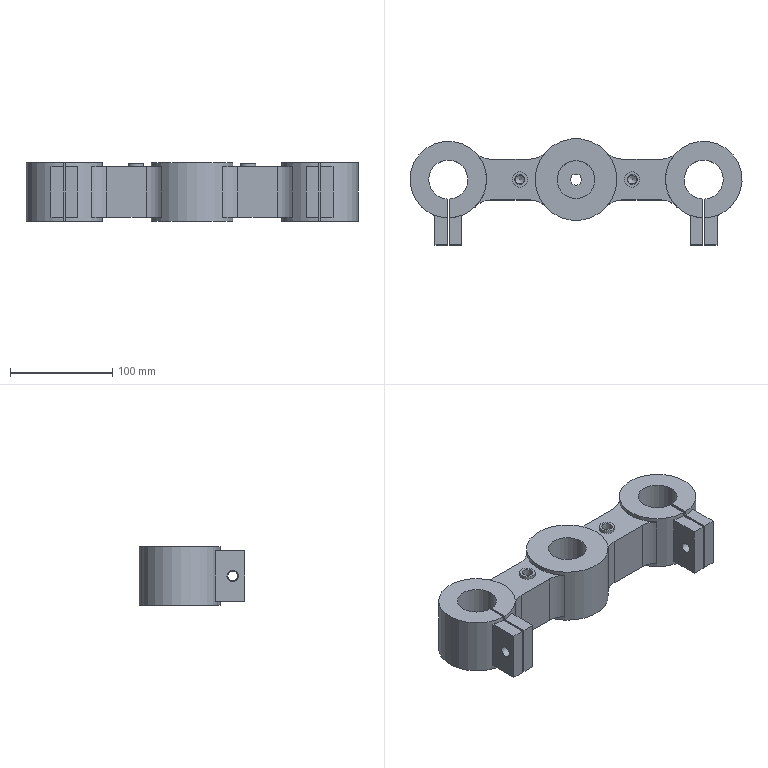Component | NX | PRESS_PLATE | 1 solid | 68 faces | volume 890602 mm3 | plane 40 | cylinder 24 | cone 4 | commonest cylinder face diameters 40 x8 75 x2 38.2 x2 10.5 x2 15 x2 10 x2 9.732 x2 80 x1